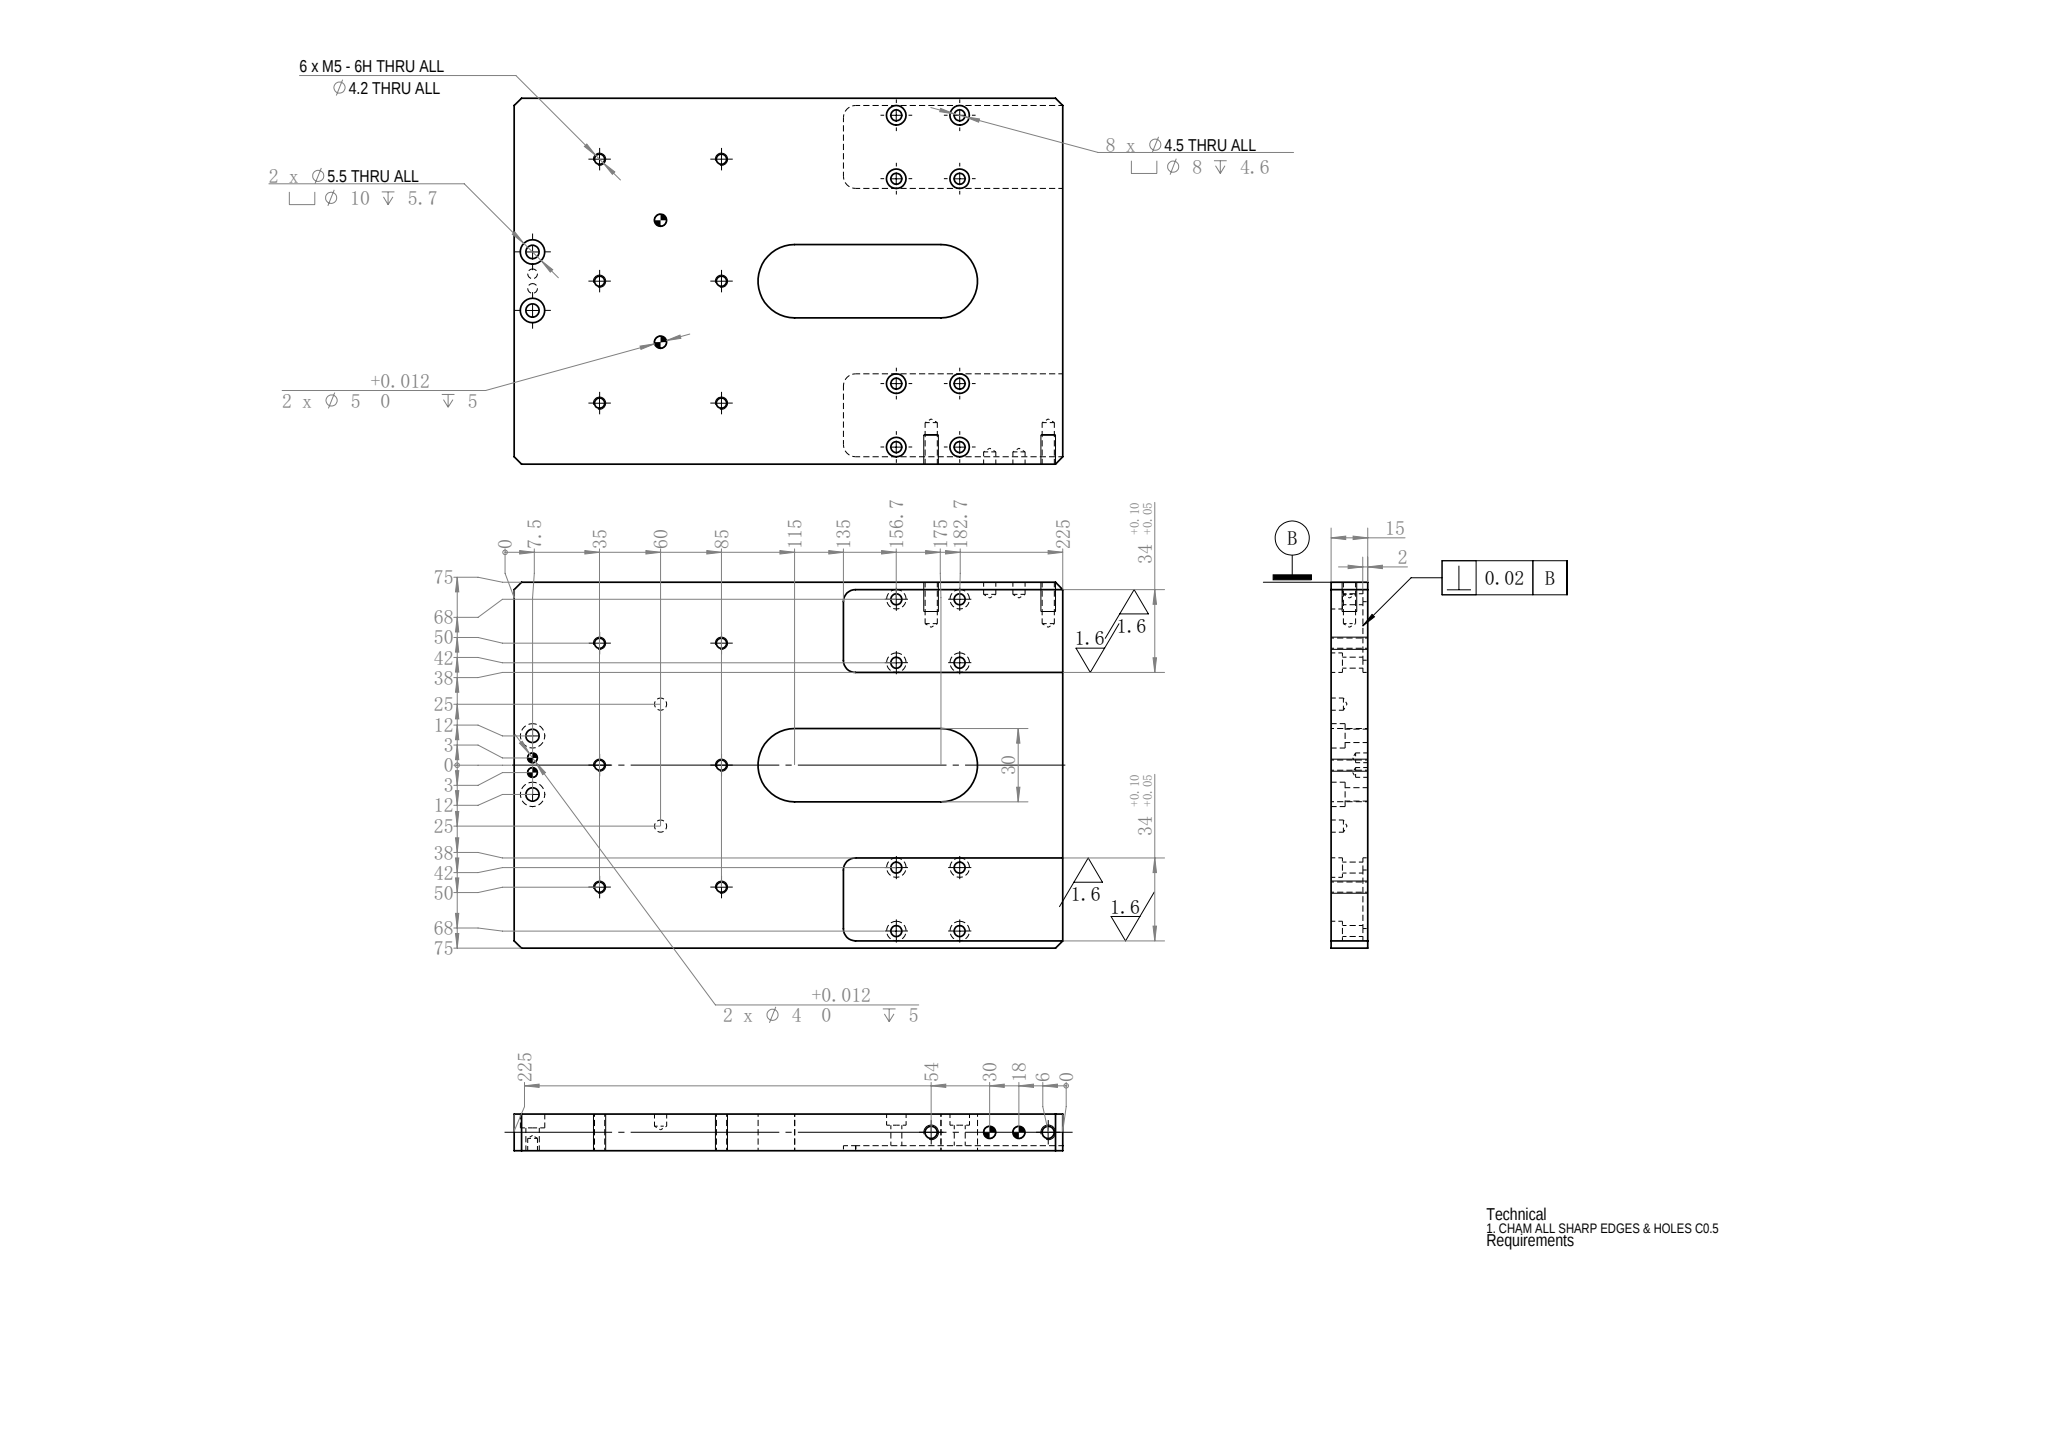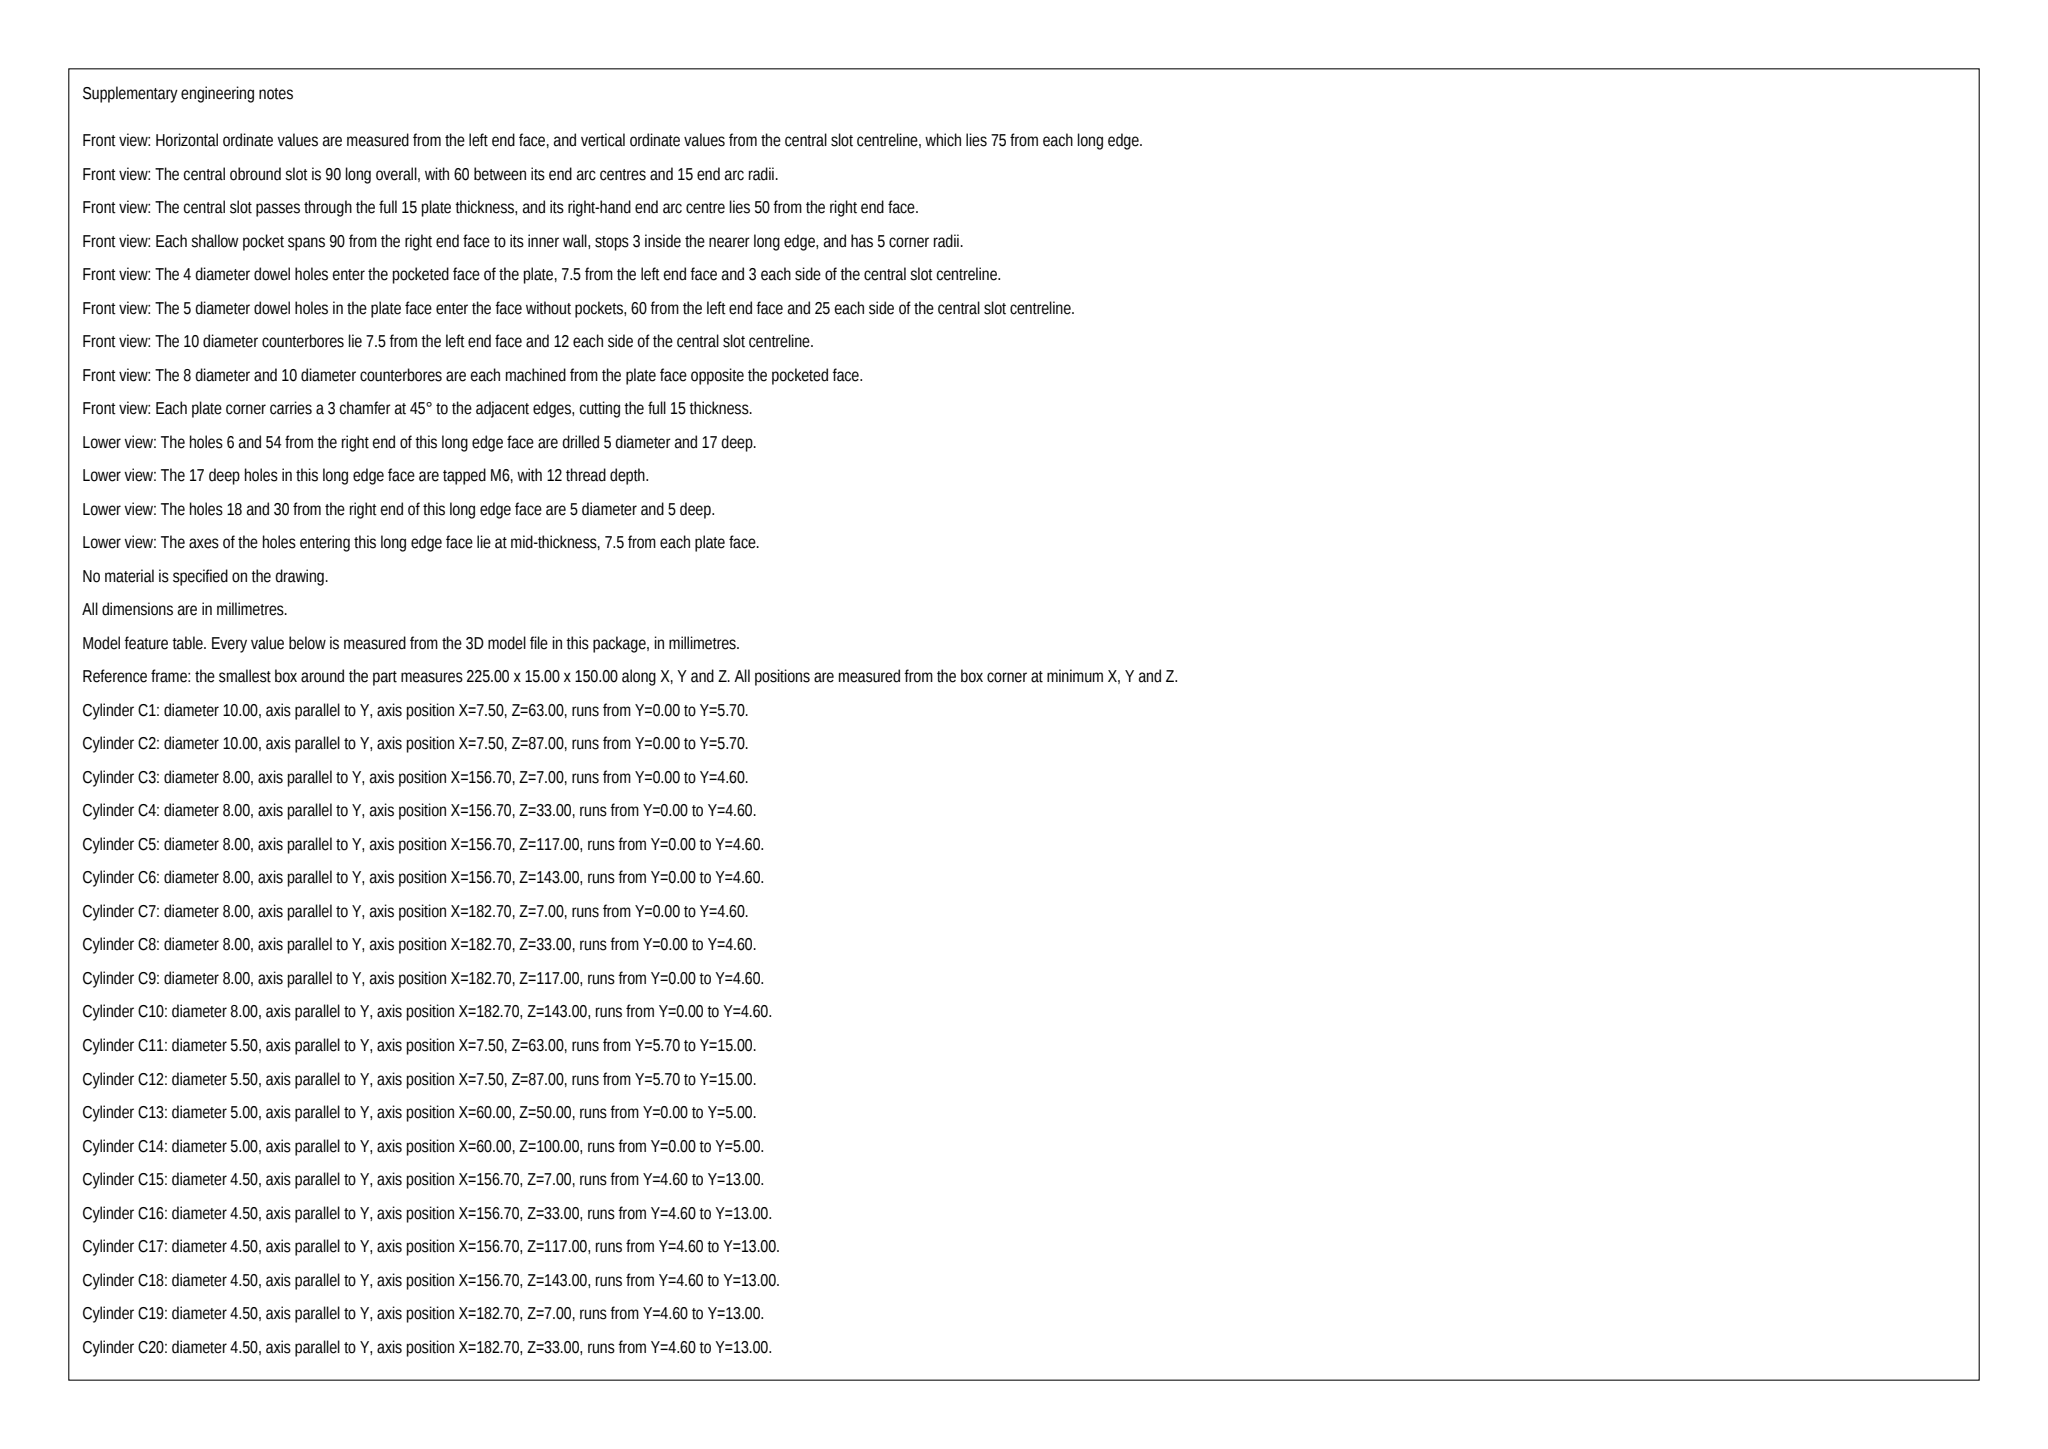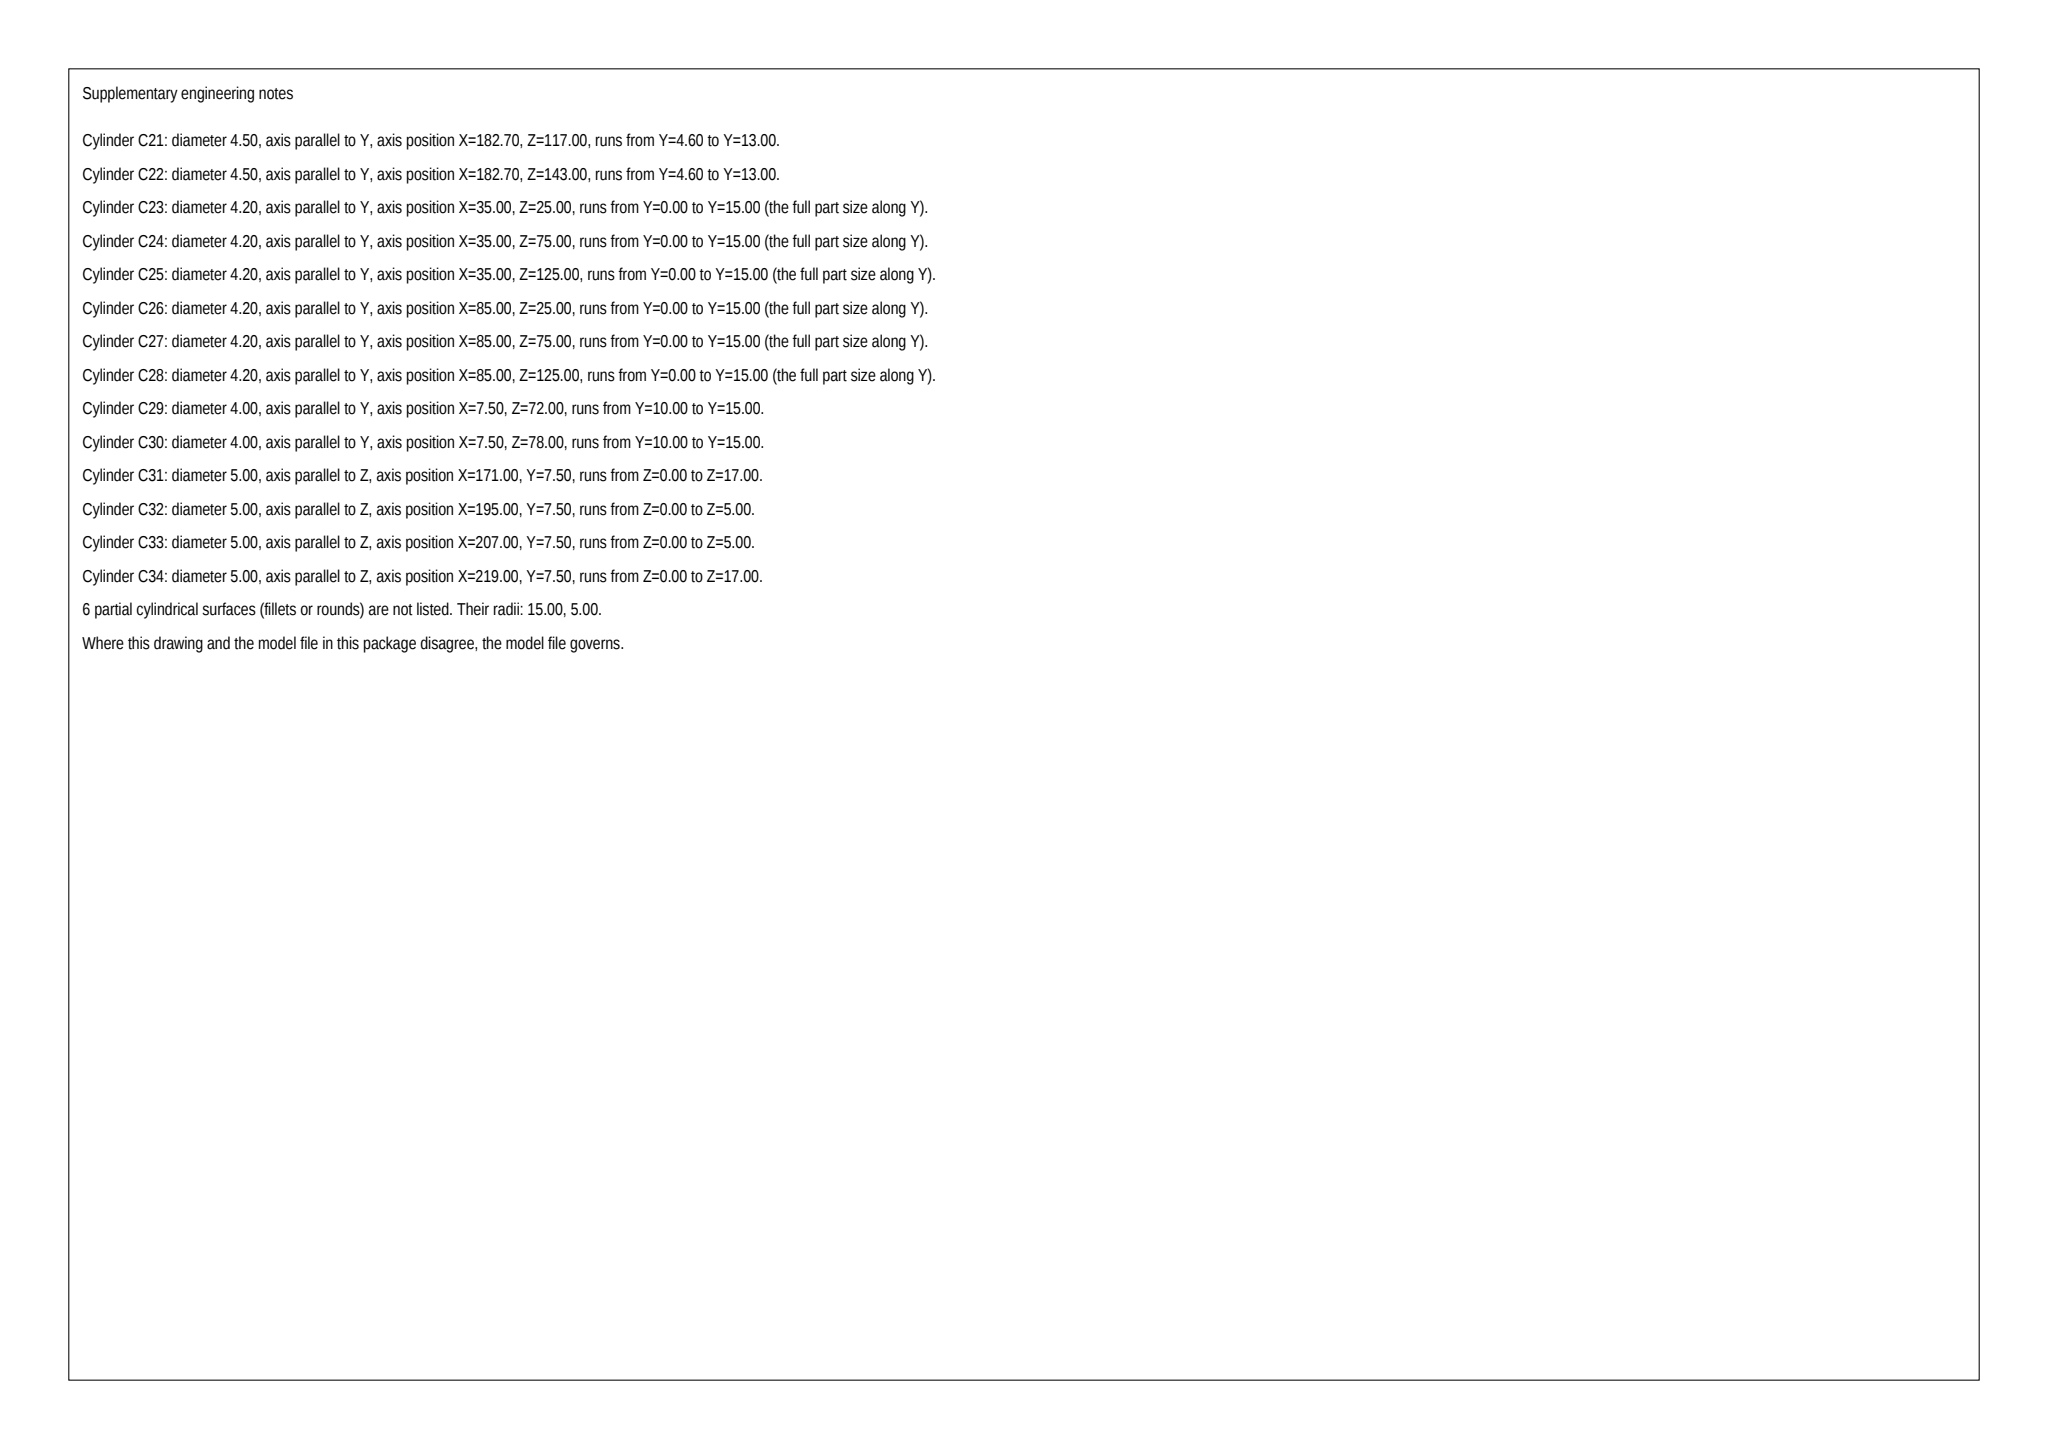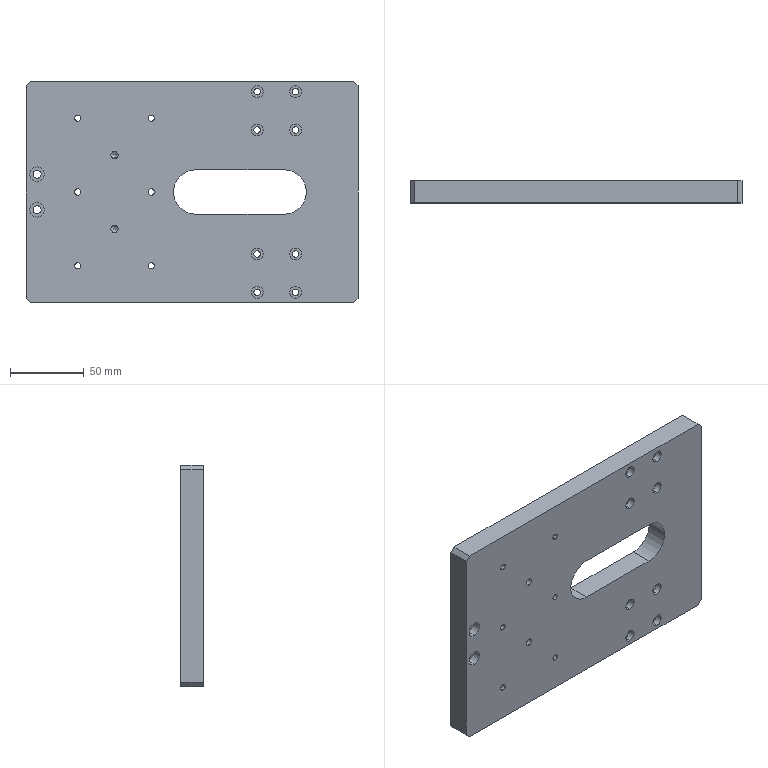Part | SolidWorks | mm | 1 solid | 120 faces | box 225 x 15 x 150 mm | volume 449422 mm3 | cylinder 74 | plane 30 | cone 16 | commonest cylinder face diameters 8 x16 4.5 x16 5 x12 4.2 x12 10 x8 4 x4 5.5 x4 30 x2
Drawing notes:
END-FACE HOLES: 8 x Ø5, IN BOTH 15 THK ENDS, ON ¢ 7.5 FROM BACK | from the solid: Ø5 cyls, axis z, at x=171/195/207/219, y=7.5; each count 2 (z=0 & z=150 faces)
Ø5 AT 54 & 6 FROM END DP 17; Ø5 AT 30 & 18 FROM END DP 5 | from the solid: Ø5 axis-z lengths: 17 at x=171 (225-54) & x=219 (225-6); 5 at x=195 (225-30) & x=207 (225-18)
END-FACE Ø5 HOLES: 4 PER END, TYP BOTH ENDS, 8 TOTAL | from the solid: each Ø5 axis-z cylinder listed with count 2, i.e. mirrored on z=0 and z=150 faces
4 x Ø10 (R5) DP 2 CORNER RELIEF AT 140, ±43 & ±67 FROM ¢ | from the solid: Ø10 axis-y cyls, L=2, at x=140, z=8/32/118/142 (center z=75) in 2 deep pockets (z planes 3,37,113,147)
build123d program:
from build123d import *

# Parameters (mm, degrees)
SKETCH1_W                                           = 225
SKETCH1_H                                           = 150
BOSS_EXTRUDE1_DEPTH                                 = 7.5
HOLE_SIZE_ACCORDING_TO_TYPE_1_OF_SLOTTE_D           = 4.5
HOLE_SIZE_ACCORDING_TO_TYPE_1_OF_SLOTTE_CBORE_D     = 8
HOLE_SIZE_ACCORDING_TO_TYPE_1_OF_SLOTTE_CBORE_DEPTH = 4.6
CUT_EXTRUDE1_DEPTH                                  = 2
CHAMFER1_SIZE                                       = 3
HOLE_SIZE_ACCORDING_TO_TYPE_1_OF_HEXAGO_D           = 5.5
HOLE_SIZE_ACCORDING_TO_TYPE_1_OF_HEXAGO_CBORE_D     = 10
HOLE_SIZE_ACCORDING_TO_TYPE_1_OF_HEXAGO_CBORE_DEPTH = 5.7
M5_TAPPED_HOLE1_D                                   = 4.2
SIZE_MM_DOWEL_PIN_HOLE_1_D                          = 4
SIZE_MM_DOWEL_PIN_HOLE_1_DEPTH                      = 5
SIZE_MM_DOWEL_PIN_HOLE_1_TIP                        = 1.202
SIZE_MM_DOWEL_PIN_HOLE_2_D                          = 5
SIZE_MM_DOWEL_PIN_HOLE_2_DEPTH                      = 5
SIZE_MM_DOWEL_PIN_HOLE_2_TIP                        = 1.502
CUT_EXTRUDE2_DEPTH                                  = 137.038
SIZE_MM_DOWEL_PIN_HOLE_3_D                          = 5
SIZE_MM_DOWEL_PIN_HOLE_3_DEPTH                      = 5
SIZE_MM_DOWEL_PIN_HOLE_3_TIP                        = 1.502
M6_TAPPED_HOLE1_D                                   = 5
M6_TAPPED_HOLE1_DEPTH                               = 17
M6_TAPPED_HOLE1_TIP                                 = 1.502


with BuildPart() as part:
    # Sketch1 → Boss-Extrude1 (new, symmetric)
    with BuildSketch(Plane(origin=(0, 0, 0), x_dir=(1, 0, 0), z_dir=(0, 1, 0))):
        Rectangle(SKETCH1_W, SKETCH1_H)
    extrude(amount=BOSS_EXTRUDE1_DEPTH, both=True)

    # Hole Size_According to_ Type 1 of Slotte (through all)
    with Locations(Plane(origin=(0, -7.5, 0), x_dir=(-1, 0, 0), z_dir=(0, -1, 0))):
        with Locations((-44.2, 42), (-44.2, 68), (-70.2, 42), (-70.2, 68)):
            hole_size_according_to_type_1_of_slotte = CounterBoreHole(HOLE_SIZE_ACCORDING_TO_TYPE_1_OF_SLOTTE_D / 2, HOLE_SIZE_ACCORDING_TO_TYPE_1_OF_SLOTTE_CBORE_D / 2, HOLE_SIZE_ACCORDING_TO_TYPE_1_OF_SLOTTE_CBORE_DEPTH)

    # Sketch5 → Cut-Extrude1 (cut)
    with BuildSketch(Plane(origin=(0, 7.5, 0), x_dir=(1, 0, 0), z_dir=(0, 1, 0))):
        with BuildLine():
            Line((112.5, 72), (27.5, 72))
            ThreePointArc((27.5, 72), (23.964, 70.536), (22.5, 67))
            Line((22.5, 67), (22.5, 43))
            ThreePointArc((22.5, 43), (23.964, 39.464), (27.5, 38))
            Line((27.5, 38), (112.5, 38))
            Line((112.5, 38), (112.5, 72))
        make_face()
    cut_extrude1 = extrude(amount=-CUT_EXTRUDE1_DEPTH, mode=Mode.SUBTRACT)

    # Mirror1: Hole Size_According to_ Type 1 of Slotte, Cut-Extrude1 across plane
    add(hole_size_according_to_type_1_of_slotte.mirror(Plane.XY), mode=Mode.SUBTRACT)
    add(cut_extrude1.mirror(Plane.XY), mode=Mode.SUBTRACT)

    # Chamfer1
    chamfer1_edges = [part.edges().sort_by_distance(p)[0] for p in [
        (112.5, 0, -75),
        (-112.5, 0, -75),
        (-112.5, 0, 75),
        (112.5, 0, 75),
    ]]
    chamfer(chamfer1_edges, length=CHAMFER1_SIZE)

    # Hole Size_According to_ Type 1 of Hexago (through all)
    with Locations(Plane(origin=(0, -7.5, 0), x_dir=(-1, 0, 0), z_dir=(0, -1, 0))):
        with Locations((105, 12), (105, -12)):
            CounterBoreHole(HOLE_SIZE_ACCORDING_TO_TYPE_1_OF_HEXAGO_D / 2, HOLE_SIZE_ACCORDING_TO_TYPE_1_OF_HEXAGO_CBORE_D / 2, HOLE_SIZE_ACCORDING_TO_TYPE_1_OF_HEXAGO_CBORE_DEPTH)

    # M5 Tapped Hole1 (through all)
    with Locations(Plane(origin=(0, -7.5, 0), x_dir=(-1, 0, 0), z_dir=(0, -1, 0))):
        with Locations((77.5, 0), (77.5, -50), (77.5, 50), (27.5, 50), (27.5, 0), (27.5, -50)):
            Hole(M5_TAPPED_HOLE1_D / 2)

    # Size mm Dowel Pin Hole 1
    with Locations(Plane(origin=(0, 7.5, 0), x_dir=(1, 0, 0), z_dir=(0, 1, 0))):
        with Locations((-105, 3), (-105, -3)):
            Hole(SIZE_MM_DOWEL_PIN_HOLE_1_D / 2, depth=SIZE_MM_DOWEL_PIN_HOLE_1_DEPTH)
            with Locations((0, 0, -(SIZE_MM_DOWEL_PIN_HOLE_1_DEPTH + SIZE_MM_DOWEL_PIN_HOLE_1_TIP / 2))):  # 118° drill point
                Cone(0, SIZE_MM_DOWEL_PIN_HOLE_1_D / 2, SIZE_MM_DOWEL_PIN_HOLE_1_TIP, mode=Mode.SUBTRACT)

    # Size mm Dowel Pin Hole 2
    with Locations(Plane(origin=(0, -7.5, 0), x_dir=(-1, 0, 0), z_dir=(0, -1, 0))):
        with Locations((52.5, 25), (52.5, -25)):
            Hole(SIZE_MM_DOWEL_PIN_HOLE_2_D / 2, depth=SIZE_MM_DOWEL_PIN_HOLE_2_DEPTH)
            with Locations((0, 0, -(SIZE_MM_DOWEL_PIN_HOLE_2_DEPTH + SIZE_MM_DOWEL_PIN_HOLE_2_TIP / 2))):  # 118° drill point
                Cone(0, SIZE_MM_DOWEL_PIN_HOLE_2_D / 2, SIZE_MM_DOWEL_PIN_HOLE_2_TIP, mode=Mode.SUBTRACT)

    # Sketch16 → Cut-Extrude2 (cut, through all)
    with BuildSketch(Plane.XZ.offset(7.5)):
        with BuildLine():
            Line((2.5, 15), (62.5, 15))
            ThreePointArc((62.5, 15), (77.5, 0), (62.5, -15))
            Line((62.5, -15), (2.5, -15))
            ThreePointArc((2.5, -15), (-12.5, 0), (2.5, 15))
        make_face()
    extrude(amount=-CUT_EXTRUDE2_DEPTH, mode=Mode.SUBTRACT)

    # Size mm Dowel Pin Hole 3
    with Locations(Plane(origin=(0, 0, -75), x_dir=(-1, 0, 0), z_dir=(0, 0, -1))):
        with Locations((-82.5, 0), (-94.5, 0)):
            Hole(SIZE_MM_DOWEL_PIN_HOLE_3_D / 2, depth=SIZE_MM_DOWEL_PIN_HOLE_3_DEPTH)
            with Locations((0, 0, -(SIZE_MM_DOWEL_PIN_HOLE_3_DEPTH + SIZE_MM_DOWEL_PIN_HOLE_3_TIP / 2))):  # 118° drill point
                Cone(0, SIZE_MM_DOWEL_PIN_HOLE_3_D / 2, SIZE_MM_DOWEL_PIN_HOLE_3_TIP, mode=Mode.SUBTRACT)

    # M6 Tapped Hole1
    with Locations(Plane(origin=(0, 0, -75), x_dir=(-1, 0, 0), z_dir=(0, 0, -1))):
        with Locations((-58.5, 0), (-106.5, 0)):
            Hole(M6_TAPPED_HOLE1_D / 2, depth=M6_TAPPED_HOLE1_DEPTH)
            with Locations((0, 0, -(M6_TAPPED_HOLE1_DEPTH + M6_TAPPED_HOLE1_TIP / 2))):  # 118° drill point
                Cone(0, M6_TAPPED_HOLE1_D / 2, M6_TAPPED_HOLE1_TIP, mode=Mode.SUBTRACT)


solid = part.part